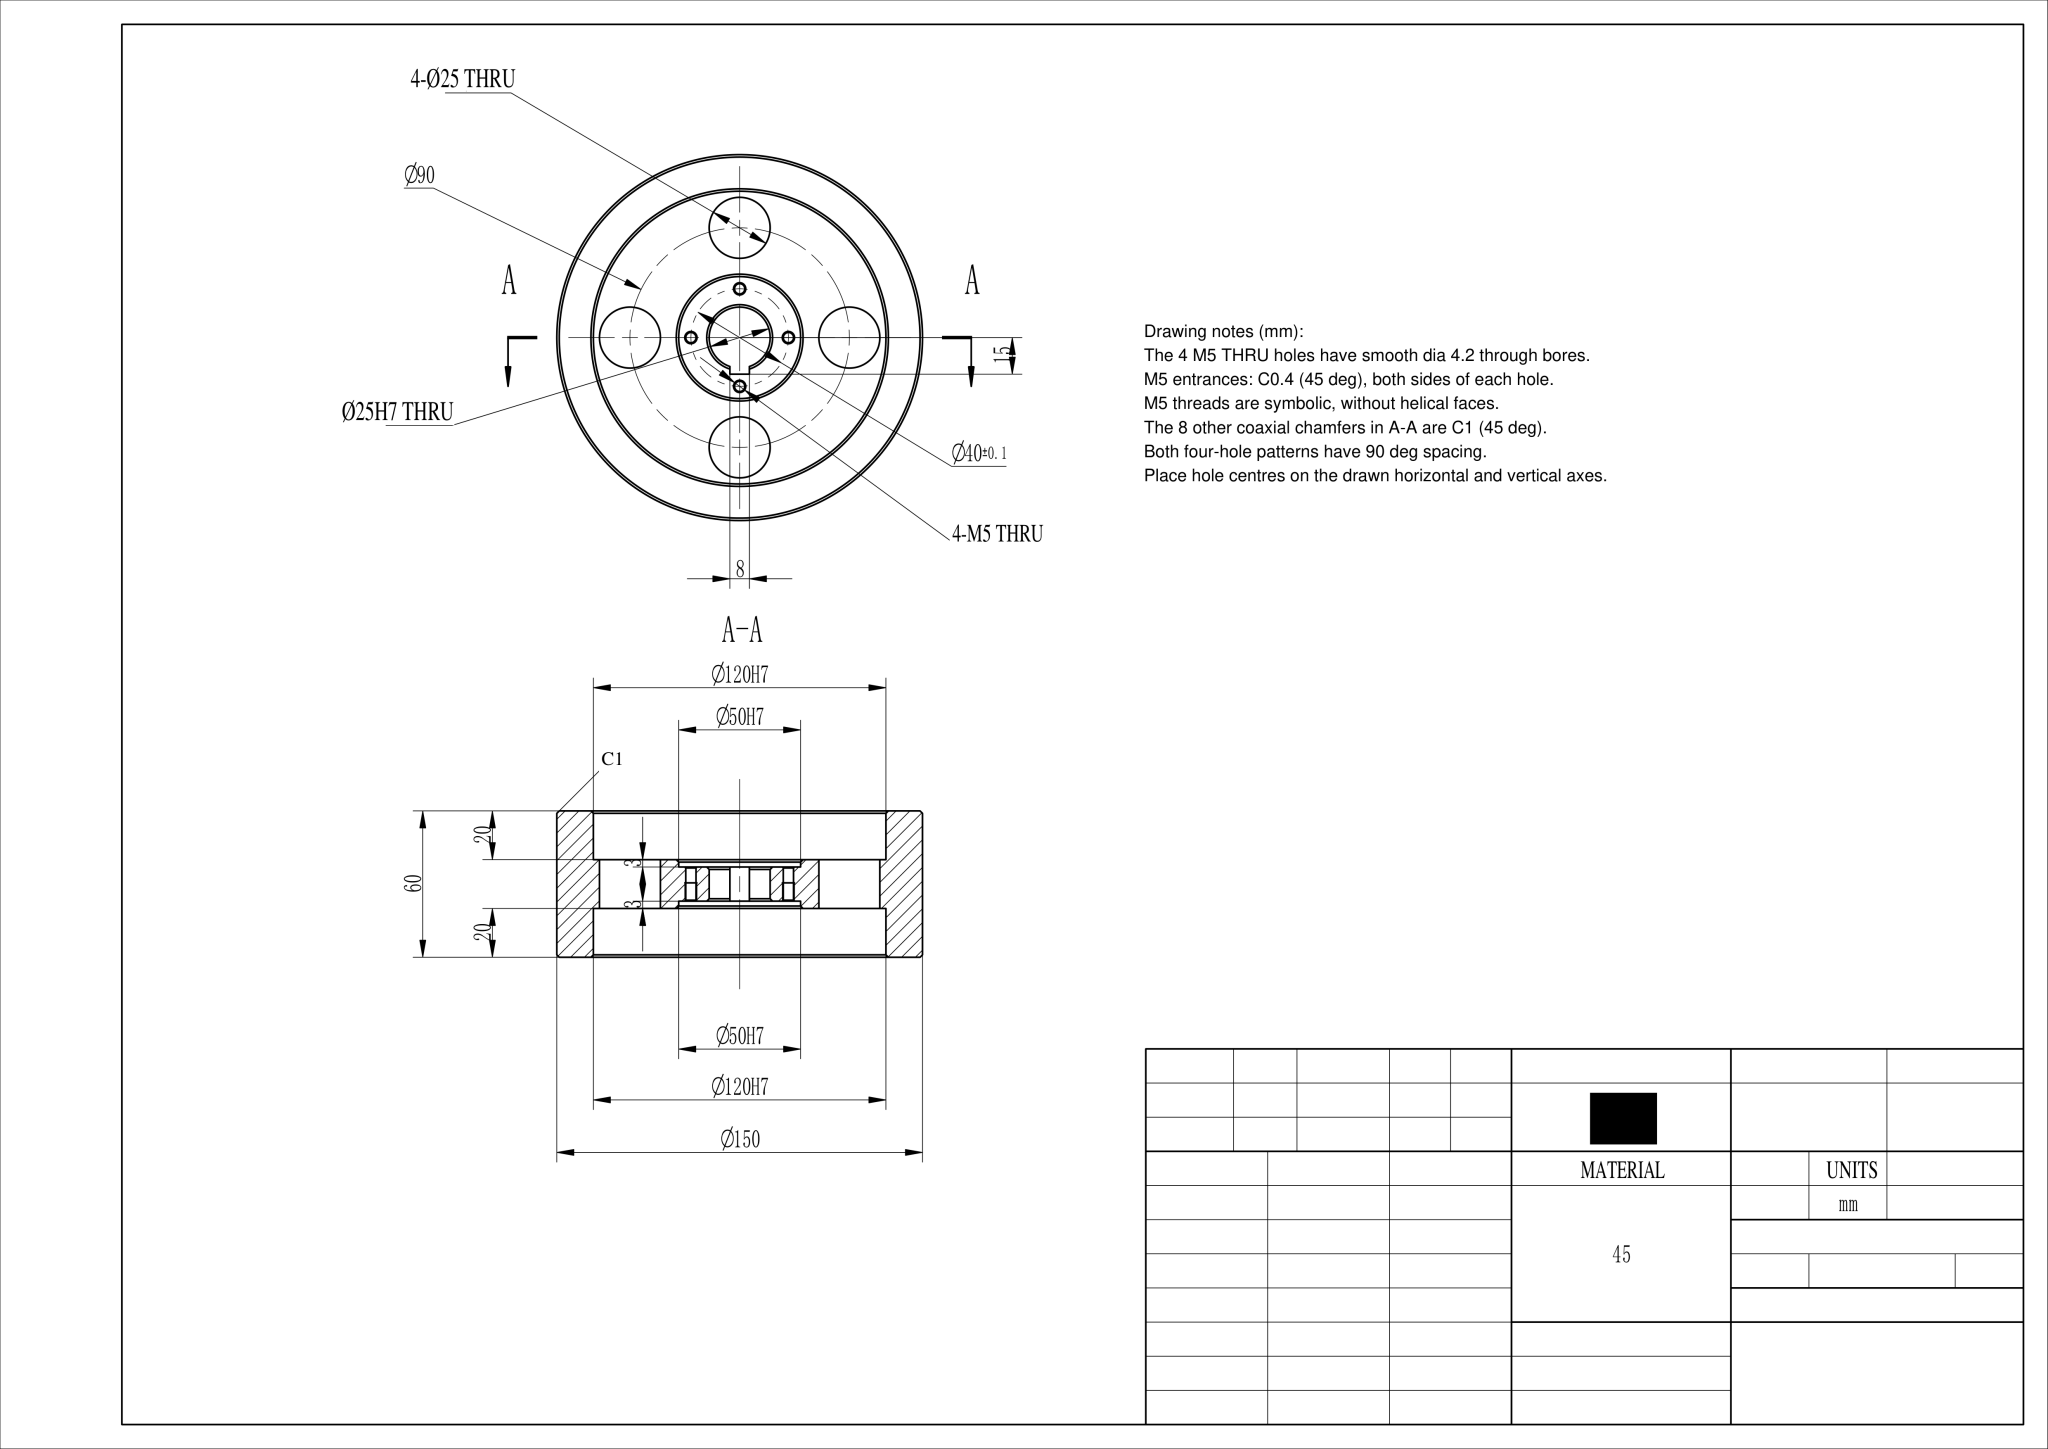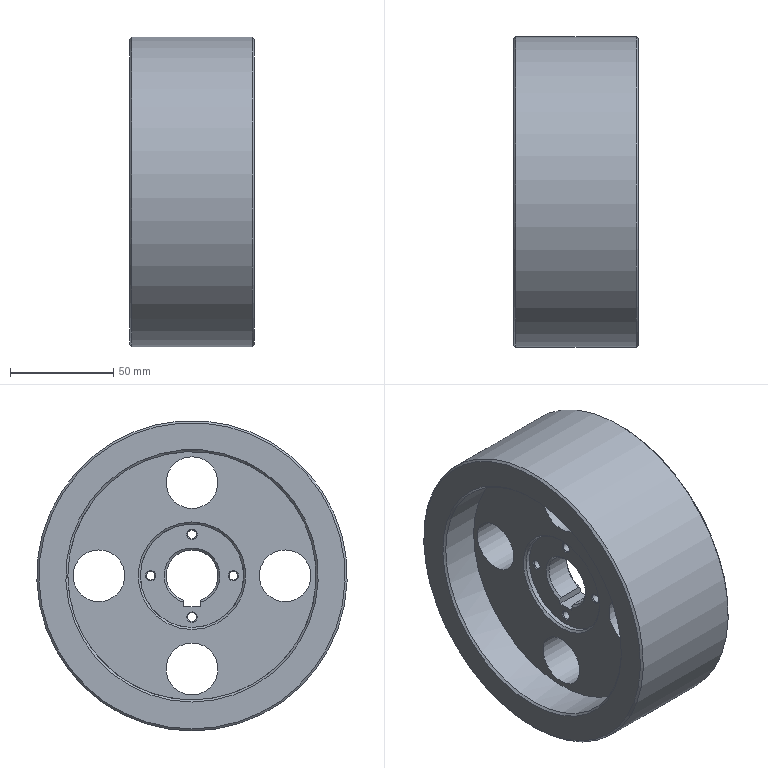Part | NX | mm | 1 solid | 39 faces | box 60 x 150 x 150 mm | volume 547806 mm3 | cone 16 | cylinder 14 | plane 9 | commonest cylinder face diameters 25 x5 4.2 x4 120 x2 50 x2 150 x1
STEP:
#1=CARTESIAN_POINT('',(0.,0.,0.));
#2=DIRECTION('',(0.,0.,1.));
#3=DIRECTION('',(1.,0.,0.));
#4=AXIS2_PLACEMENT_3D('',#1,#2,#3);
#5=(LENGTH_UNIT()NAMED_UNIT(*)SI_UNIT(.MILLI.,.METRE.));
#6=UNCERTAINTY_MEASURE_WITH_UNIT(LENGTH_MEASURE(0.0508),#5,'','');
#7=(NAMED_UNIT(*)PLANE_ANGLE_UNIT()SI_UNIT($,.RADIAN.));
#8=PLANE_ANGLE_MEASURE_WITH_UNIT(PLANE_ANGLE_MEASURE(0.01745),#7);
#9=DIMENSIONAL_EXPONENTS(0.,0.,0.,0.,0.,0.,0.);
#10=(CONVERSION_BASED_UNIT('',#8)NAMED_UNIT(#9)PLANE_ANGLE_UNIT());
#11=(NAMED_UNIT(*)SI_UNIT($,.STERADIAN.)SOLID_ANGLE_UNIT());
#12=(GEOMETRIC_REPRESENTATION_CONTEXT(3)GLOBAL_UNCERTAINTY_ASSIGNED_CONTEXT((#6))GLOBAL_UNIT_ASSIGNED_CONTEXT((#5,#10,#11))REPRESENTATION_CONTEXT('',''));
#13=SHAPE_REPRESENTATION('',(#4),#12);
#14=CARTESIAN_POINT('',(-29.,0.,-75.));
#15=VERTEX_POINT('',#14);
#16=CARTESIAN_POINT('',(-29.,0.,0.));
#17=DIRECTION('',(1.,0.,0.));
#18=DIRECTION('',(0.,0.,-1.));
#19=AXIS2_PLACEMENT_3D('',#16,#17,#18);
#20=CIRCLE('',#19,75.);
#21=EDGE_CURVE('',#15,#15,#20,.T.);
#22=ORIENTED_EDGE('',*,*,#21,.T.);
#23=EDGE_LOOP('',(#22));
#24=FACE_BOUND('',#23,.T.);
#25=CARTESIAN_POINT('',(29.,0.,-75.));
#26=VERTEX_POINT('',#25);
#27=CARTESIAN_POINT('',(29.,0.,0.));
#28=DIRECTION('',(-1.,0.,0.));
#29=DIRECTION('',(0.,0.,-1.));
#30=AXIS2_PLACEMENT_3D('',#27,#28,#29);
#31=CIRCLE('',#30,75.);
#32=EDGE_CURVE('',#26,#26,#31,.T.);
#33=ORIENTED_EDGE('',*,*,#32,.T.);
#34=EDGE_LOOP('',(#33));
#35=FACE_BOUND('',#34,.T.);
#36=CARTESIAN_POINT('',(30.,0.,0.));
#37=DIRECTION('',(-1.,0.,0.));
#38=DIRECTION('',(0.,0.,1.));
#39=AXIS2_PLACEMENT_3D('',#36,#37,#38);
#40=CYLINDRICAL_SURFACE('',#39,75.);
#41=ADVANCED_FACE('',(#24,#35),#40,.T.);
#42=CARTESIAN_POINT('',(30.,0.,-61.));
#43=VERTEX_POINT('',#42);
#44=CARTESIAN_POINT('',(30.,0.,0.));
#45=DIRECTION('',(-1.,0.,0.));
#46=DIRECTION('',(0.,0.,-1.));
#47=AXIS2_PLACEMENT_3D('',#44,#45,#46);
#48=CIRCLE('',#47,61.);
#49=EDGE_CURVE('',#43,#43,#48,.T.);
#50=ORIENTED_EDGE('',*,*,#49,.T.);
#51=EDGE_LOOP('',(#50));
#52=FACE_BOUND('',#51,.T.);
#53=CARTESIAN_POINT('',(30.,0.,-74.));
#54=VERTEX_POINT('',#53);
#55=CARTESIAN_POINT('',(30.,0.,0.));
#56=DIRECTION('',(1.,0.,0.));
#57=DIRECTION('',(0.,0.,-1.));
#58=AXIS2_PLACEMENT_3D('',#55,#56,#57);
#59=CIRCLE('',#58,74.);
#60=EDGE_CURVE('',#54,#54,#59,.T.);
#61=ORIENTED_EDGE('',*,*,#60,.T.);
#62=EDGE_LOOP('',(#61));
#63=FACE_BOUND('',#62,.T.);
#64=CARTESIAN_POINT('',(30.,0.,0.));
#65=DIRECTION('',(1.,0.,0.));
#66=DIRECTION('',(0.,0.,-1.));
#67=AXIS2_PLACEMENT_3D('',#64,#65,#66);
#68=PLANE('',#67);
#69=ADVANCED_FACE('',(#52,#63),#68,.T.);
#70=CARTESIAN_POINT('',(-30.,0.,-61.));
#71=VERTEX_POINT('',#70);
#72=CARTESIAN_POINT('',(-30.,0.,0.));
#73=DIRECTION('',(1.,0.,0.));
#74=DIRECTION('',(0.,0.,-1.));
#75=AXIS2_PLACEMENT_3D('',#72,#73,#74);
#76=CIRCLE('',#75,61.);
#77=EDGE_CURVE('',#71,#71,#76,.T.);
#78=ORIENTED_EDGE('',*,*,#77,.T.);
#79=EDGE_LOOP('',(#78));
#80=FACE_BOUND('',#79,.T.);
#81=CARTESIAN_POINT('',(-30.,0.,-74.));
#82=VERTEX_POINT('',#81);
#83=CARTESIAN_POINT('',(-30.,0.,0.));
#84=DIRECTION('',(-1.,0.,0.));
#85=DIRECTION('',(0.,0.,-1.));
#86=AXIS2_PLACEMENT_3D('',#83,#84,#85);
#87=CIRCLE('',#86,74.);
#88=EDGE_CURVE('',#82,#82,#87,.T.);
#89=ORIENTED_EDGE('',*,*,#88,.T.);
#90=EDGE_LOOP('',(#89));
#91=FACE_BOUND('',#90,.T.);
#92=CARTESIAN_POINT('',(-30.,0.,0.));
#93=DIRECTION('',(1.,0.,0.));
#94=DIRECTION('',(0.,0.,-1.));
#95=AXIS2_PLACEMENT_3D('',#92,#93,#94);
#96=PLANE('',#95);
#97=ADVANCED_FACE('',(#80,#91),#96,.F.);
#98=CARTESIAN_POINT('',(29.,0.,-60.));
#99=VERTEX_POINT('',#98);
#100=CARTESIAN_POINT('',(29.,0.,0.));
#101=DIRECTION('',(1.,0.,0.));
#102=DIRECTION('',(0.,0.,-1.));
#103=AXIS2_PLACEMENT_3D('',#100,#101,#102);
#104=CIRCLE('',#103,60.);
#105=EDGE_CURVE('',#99,#99,#104,.T.);
#106=ORIENTED_EDGE('',*,*,#105,.T.);
#107=EDGE_LOOP('',(#106));
#108=FACE_BOUND('',#107,.T.);
#109=CARTESIAN_POINT('',(10.,60.,-0.));
#110=VERTEX_POINT('',#109);
#111=CARTESIAN_POINT('',(10.,0.,0.));
#112=DIRECTION('',(-1.,0.,0.));
#113=DIRECTION('',(0.,1.,-0.));
#114=AXIS2_PLACEMENT_3D('',#111,#112,#113);
#115=CIRCLE('',#114,60.);
#116=EDGE_CURVE('',#110,#110,#115,.T.);
#117=ORIENTED_EDGE('',*,*,#116,.T.);
#118=EDGE_LOOP('',(#117));
#119=FACE_BOUND('',#118,.T.);
#120=CARTESIAN_POINT('',(10.,0.,0.));
#121=DIRECTION('',(1.,0.,0.));
#122=DIRECTION('',(0.,0.,-1.));
#123=AXIS2_PLACEMENT_3D('',#120,#121,#122);
#124=CYLINDRICAL_SURFACE('',#123,60.);
#125=ADVANCED_FACE('',(#108,#119),#124,.F.);
#126=CARTESIAN_POINT('',(10.,0.,-26.));
#127=VERTEX_POINT('',#126);
#128=CARTESIAN_POINT('',(10.,0.,0.));
#129=DIRECTION('',(-1.,0.,0.));
#130=DIRECTION('',(0.,0.,-1.));
#131=AXIS2_PLACEMENT_3D('',#128,#129,#130);
#132=CIRCLE('',#131,26.);
#133=EDGE_CURVE('',#127,#127,#132,.T.);
#134=ORIENTED_EDGE('',*,*,#133,.T.);
#135=EDGE_LOOP('',(#134));
#136=FACE_BOUND('',#135,.T.);
#137=CARTESIAN_POINT('',(10.,-45.,12.5));
#138=VERTEX_POINT('',#137);
#139=CARTESIAN_POINT('',(10.,-45.,-0.));
#140=DIRECTION('',(-1.,0.,0.));
#141=DIRECTION('',(0.,0.,1.));
#142=AXIS2_PLACEMENT_3D('',#139,#140,#141);
#143=CIRCLE('',#142,12.5);
#144=EDGE_CURVE('',#138,#138,#143,.T.);
#145=ORIENTED_EDGE('',*,*,#144,.T.);
#146=EDGE_LOOP('',(#145));
#147=FACE_BOUND('',#146,.T.);
#148=CARTESIAN_POINT('',(10.,0.,-32.5));
#149=VERTEX_POINT('',#148);
#150=CARTESIAN_POINT('',(10.,0.,-45.));
#151=DIRECTION('',(-1.,0.,0.));
#152=DIRECTION('',(0.,0.,1.));
#153=AXIS2_PLACEMENT_3D('',#150,#151,#152);
#154=CIRCLE('',#153,12.5);
#155=EDGE_CURVE('',#149,#149,#154,.T.);
#156=ORIENTED_EDGE('',*,*,#155,.T.);
#157=EDGE_LOOP('',(#156));
#158=FACE_BOUND('',#157,.T.);
#159=CARTESIAN_POINT('',(10.,45.,12.5));
#160=VERTEX_POINT('',#159);
#161=CARTESIAN_POINT('',(10.,45.,0.));
#162=DIRECTION('',(-1.,0.,0.));
#163=DIRECTION('',(0.,0.,1.));
#164=AXIS2_PLACEMENT_3D('',#161,#162,#163);
#165=CIRCLE('',#164,12.5);
#166=EDGE_CURVE('',#160,#160,#165,.T.);
#167=ORIENTED_EDGE('',*,*,#166,.T.);
#168=EDGE_LOOP('',(#167));
#169=FACE_BOUND('',#168,.T.);
#170=CARTESIAN_POINT('',(10.,0.,57.5));
#171=VERTEX_POINT('',#170);
#172=CARTESIAN_POINT('',(10.,0.,45.));
#173=DIRECTION('',(-1.,0.,0.));
#174=DIRECTION('',(0.,0.,1.));
#175=AXIS2_PLACEMENT_3D('',#172,#173,#174);
#176=CIRCLE('',#175,12.5);
#177=EDGE_CURVE('',#171,#171,#176,.T.);
#178=ORIENTED_EDGE('',*,*,#177,.T.);
#179=EDGE_LOOP('',(#178));
#180=FACE_BOUND('',#179,.T.);
#181=ORIENTED_EDGE('',*,*,#116,.F.);
#182=EDGE_LOOP('',(#181));
#183=FACE_BOUND('',#182,.T.);
#184=CARTESIAN_POINT('',(10.,0.,0.));
#185=DIRECTION('',(1.,0.,0.));
#186=DIRECTION('',(0.,0.,-1.));
#187=AXIS2_PLACEMENT_3D('',#184,#185,#186);
#188=PLANE('',#187);
#189=ADVANCED_FACE('',(#136,#147,#158,#169,#180,#183),#188,.T.);
#190=CARTESIAN_POINT('',(-29.,0.,-60.));
#191=VERTEX_POINT('',#190);
#192=CARTESIAN_POINT('',(-29.,0.,0.));
#193=DIRECTION('',(-1.,0.,0.));
#194=DIRECTION('',(0.,0.,-1.));
#195=AXIS2_PLACEMENT_3D('',#192,#193,#194);
#196=CIRCLE('',#195,60.);
#197=EDGE_CURVE('',#191,#191,#196,.T.);
#198=ORIENTED_EDGE('',*,*,#197,.T.);
#199=EDGE_LOOP('',(#198));
#200=FACE_BOUND('',#199,.T.);
#201=CARTESIAN_POINT('',(-10.,60.,-0.));
#202=VERTEX_POINT('',#201);
#203=CARTESIAN_POINT('',(-10.,0.,0.));
#204=DIRECTION('',(-1.,0.,0.));
#205=DIRECTION('',(0.,1.,-0.));
#206=AXIS2_PLACEMENT_3D('',#203,#204,#205);
#207=CIRCLE('',#206,60.);
#208=EDGE_CURVE('',#202,#202,#207,.T.);
#209=ORIENTED_EDGE('',*,*,#208,.F.);
#210=EDGE_LOOP('',(#209));
#211=FACE_BOUND('',#210,.T.);
#212=CARTESIAN_POINT('',(-10.,0.,0.));
#213=DIRECTION('',(-1.,0.,0.));
#214=DIRECTION('',(0.,0.,1.));
#215=AXIS2_PLACEMENT_3D('',#212,#213,#214);
#216=CYLINDRICAL_SURFACE('',#215,60.);
#217=ADVANCED_FACE('',(#200,#211),#216,.F.);
#218=CARTESIAN_POINT('',(-10.,0.,-26.));
#219=VERTEX_POINT('',#218);
#220=CARTESIAN_POINT('',(-10.,0.,0.));
#221=DIRECTION('',(1.,0.,0.));
#222=DIRECTION('',(0.,0.,-1.));
#223=AXIS2_PLACEMENT_3D('',#220,#221,#222);
#224=CIRCLE('',#223,26.);
#225=EDGE_CURVE('',#219,#219,#224,.T.);
#226=ORIENTED_EDGE('',*,*,#225,.T.);
#227=EDGE_LOOP('',(#226));
#228=FACE_BOUND('',#227,.T.);
#229=CARTESIAN_POINT('',(-10.,-45.,-12.5));
#230=VERTEX_POINT('',#229);
#231=CARTESIAN_POINT('',(-10.,-45.,-0.));
#232=DIRECTION('',(1.,0.,0.));
#233=DIRECTION('',(0.,0.,-1.));
#234=AXIS2_PLACEMENT_3D('',#231,#232,#233);
#235=CIRCLE('',#234,12.5);
#236=EDGE_CURVE('',#230,#230,#235,.T.);
#237=ORIENTED_EDGE('',*,*,#236,.T.);
#238=EDGE_LOOP('',(#237));
#239=FACE_BOUND('',#238,.T.);
#240=CARTESIAN_POINT('',(-10.,0.,-57.5));
#241=VERTEX_POINT('',#240);
#242=CARTESIAN_POINT('',(-10.,0.,-45.));
#243=DIRECTION('',(1.,0.,0.));
#244=DIRECTION('',(0.,0.,-1.));
#245=AXIS2_PLACEMENT_3D('',#242,#243,#244);
#246=CIRCLE('',#245,12.5);
#247=EDGE_CURVE('',#241,#241,#246,.T.);
#248=ORIENTED_EDGE('',*,*,#247,.T.);
#249=EDGE_LOOP('',(#248));
#250=FACE_BOUND('',#249,.T.);
#251=CARTESIAN_POINT('',(-10.,45.,-12.5));
#252=VERTEX_POINT('',#251);
#253=CARTESIAN_POINT('',(-10.,45.,0.));
#254=DIRECTION('',(1.,0.,0.));
#255=DIRECTION('',(0.,0.,-1.));
#256=AXIS2_PLACEMENT_3D('',#253,#254,#255);
#257=CIRCLE('',#256,12.5);
#258=EDGE_CURVE('',#252,#252,#257,.T.);
#259=ORIENTED_EDGE('',*,*,#258,.T.);
#260=EDGE_LOOP('',(#259));
#261=FACE_BOUND('',#260,.T.);
#262=CARTESIAN_POINT('',(-10.,0.,32.5));
#263=VERTEX_POINT('',#262);
#264=CARTESIAN_POINT('',(-10.,0.,45.));
#265=DIRECTION('',(1.,0.,0.));
#266=DIRECTION('',(0.,0.,-1.));
#267=AXIS2_PLACEMENT_3D('',#264,#265,#266);
#268=CIRCLE('',#267,12.5);
#269=EDGE_CURVE('',#263,#263,#268,.T.);
#270=ORIENTED_EDGE('',*,*,#269,.T.);
#271=EDGE_LOOP('',(#270));
#272=FACE_BOUND('',#271,.T.);
#273=ORIENTED_EDGE('',*,*,#208,.T.);
#274=EDGE_LOOP('',(#273));
#275=FACE_BOUND('',#274,.T.);
#276=CARTESIAN_POINT('',(-10.,0.,0.));
#277=DIRECTION('',(1.,0.,0.));
#278=DIRECTION('',(0.,0.,-1.));
#279=AXIS2_PLACEMENT_3D('',#276,#277,#278);
#280=PLANE('',#279);
#281=ADVANCED_FACE('',(#228,#239,#250,#261,#272,#275),#280,.F.);
#282=ORIENTED_EDGE('',*,*,#177,.F.);
#283=EDGE_LOOP('',(#282));
#284=FACE_BOUND('',#283,.T.);
#285=ORIENTED_EDGE('',*,*,#269,.F.);
#286=EDGE_LOOP('',(#285));
#287=FACE_BOUND('',#286,.T.);
#288=CARTESIAN_POINT('',(10.,0.,45.));
#289=DIRECTION('',(-1.,0.,0.));
#290=DIRECTION('',(0.,0.,1.));
#291=AXIS2_PLACEMENT_3D('',#288,#289,#290);
#292=CYLINDRICAL_SURFACE('',#291,12.5);
#293=ADVANCED_FACE('',(#284,#287),#292,.F.);
#294=ORIENTED_EDGE('',*,*,#166,.F.);
#295=EDGE_LOOP('',(#294));
#296=FACE_BOUND('',#295,.T.);
#297=ORIENTED_EDGE('',*,*,#258,.F.);
#298=EDGE_LOOP('',(#297));
#299=FACE_BOUND('',#298,.T.);
#300=CARTESIAN_POINT('',(10.,45.,0.));
#301=DIRECTION('',(-1.,0.,0.));
#302=DIRECTION('',(0.,0.,1.));
#303=AXIS2_PLACEMENT_3D('',#300,#301,#302);
#304=CYLINDRICAL_SURFACE('',#303,12.5);
#305=ADVANCED_FACE('',(#296,#299),#304,.F.);
#306=ORIENTED_EDGE('',*,*,#155,.F.);
#307=EDGE_LOOP('',(#306));
#308=FACE_BOUND('',#307,.T.);
#309=ORIENTED_EDGE('',*,*,#247,.F.);
#310=EDGE_LOOP('',(#309));
#311=FACE_BOUND('',#310,.T.);
#312=CARTESIAN_POINT('',(10.,0.,-45.));
#313=DIRECTION('',(-1.,0.,0.));
#314=DIRECTION('',(0.,0.,1.));
#315=AXIS2_PLACEMENT_3D('',#312,#313,#314);
#316=CYLINDRICAL_SURFACE('',#315,12.5);
#317=ADVANCED_FACE('',(#308,#311),#316,.F.);
#318=ORIENTED_EDGE('',*,*,#144,.F.);
#319=EDGE_LOOP('',(#318));
#320=FACE_BOUND('',#319,.T.);
#321=ORIENTED_EDGE('',*,*,#236,.F.);
#322=EDGE_LOOP('',(#321));
#323=FACE_BOUND('',#322,.T.);
#324=CARTESIAN_POINT('',(10.,-45.,-0.));
#325=DIRECTION('',(-1.,0.,0.));
#326=DIRECTION('',(0.,0.,1.));
#327=AXIS2_PLACEMENT_3D('',#324,#325,#326);
#328=CYLINDRICAL_SURFACE('',#327,12.5);
#329=ADVANCED_FACE('',(#320,#323),#328,.F.);
#330=CARTESIAN_POINT('',(9.,0.,-25.));
#331=VERTEX_POINT('',#330);
#332=CARTESIAN_POINT('',(9.,0.,0.));
#333=DIRECTION('',(1.,0.,0.));
#334=DIRECTION('',(0.,0.,-1.));
#335=AXIS2_PLACEMENT_3D('',#332,#333,#334);
#336=CIRCLE('',#335,25.);
#337=EDGE_CURVE('',#331,#331,#336,.T.);
#338=ORIENTED_EDGE('',*,*,#337,.T.);
#339=EDGE_LOOP('',(#338));
#340=FACE_BOUND('',#339,.T.);
#341=CARTESIAN_POINT('',(7.,25.,-0.));
#342=VERTEX_POINT('',#341);
#343=CARTESIAN_POINT('',(7.,0.,0.));
#344=DIRECTION('',(-1.,0.,0.));
#345=DIRECTION('',(0.,1.,-0.));
#346=AXIS2_PLACEMENT_3D('',#343,#344,#345);
#347=CIRCLE('',#346,25.);
#348=EDGE_CURVE('',#342,#342,#347,.T.);
#349=ORIENTED_EDGE('',*,*,#348,.T.);
#350=EDGE_LOOP('',(#349));
#351=FACE_BOUND('',#350,.T.);
#352=CARTESIAN_POINT('',(7.,0.,0.));
#353=DIRECTION('',(1.,0.,0.));
#354=DIRECTION('',(0.,0.,-1.));
#355=AXIS2_PLACEMENT_3D('',#352,#353,#354);
#356=CYLINDRICAL_SURFACE('',#355,25.);
#357=ADVANCED_FACE('',(#340,#351),#356,.F.);
#358=CARTESIAN_POINT('',(7.,4.,-15.));
#359=VERTEX_POINT('',#358);
#360=CARTESIAN_POINT('',(7.,4.,-12.894));
#361=VERTEX_POINT('',#360);
#362=CARTESIAN_POINT('',(7.,4.,0.));
#363=DIRECTION('',(0.,-0.,1.));
#364=VECTOR('',#363,1.);
#365=LINE('',#362,#364);
#366=EDGE_CURVE('',#359,#361,#365,.T.);
#367=ORIENTED_EDGE('',*,*,#366,.F.);
#368=CARTESIAN_POINT('',(7.,-4.,-15.));
#369=VERTEX_POINT('',#368);
#370=CARTESIAN_POINT('',(7.,0.,-15.));
#371=DIRECTION('',(0.,1.,0.));
#372=VECTOR('',#371,1.);
#373=LINE('',#370,#372);
#374=EDGE_CURVE('',#369,#359,#373,.T.);
#375=ORIENTED_EDGE('',*,*,#374,.F.);
#376=CARTESIAN_POINT('',(7.,-4.,-12.894));
#377=VERTEX_POINT('',#376);
#378=CARTESIAN_POINT('',(7.,-4.,0.));
#379=DIRECTION('',(0.,-0.,-1.));
#380=VECTOR('',#379,1.);
#381=LINE('',#378,#380);
#382=EDGE_CURVE('',#377,#369,#381,.T.);
#383=ORIENTED_EDGE('',*,*,#382,.F.);
#384=CARTESIAN_POINT('',(7.,0.,0.));
#385=DIRECTION('',(-1.,0.,0.));
#386=DIRECTION('',(0.,0.,-1.));
#387=AXIS2_PLACEMENT_3D('',#384,#385,#386);
#388=CIRCLE('',#387,13.5);
#389=EDGE_CURVE('',#377,#361,#388,.T.);
#390=ORIENTED_EDGE('',*,*,#389,.T.);
#391=EDGE_LOOP('',(#367,#375,#383,#390));
#392=FACE_BOUND('',#391,.T.);
#393=CARTESIAN_POINT('',(7.,-20.,-2.5));
#394=VERTEX_POINT('',#393);
#395=CARTESIAN_POINT('',(7.,-20.,0.));
#396=DIRECTION('',(-1.,0.,0.));
#397=DIRECTION('',(0.,0.,-1.));
#398=AXIS2_PLACEMENT_3D('',#395,#396,#397);
#399=CIRCLE('',#398,2.5);
#400=EDGE_CURVE('',#394,#394,#399,.T.);
#401=ORIENTED_EDGE('',*,*,#400,.T.);
#402=EDGE_LOOP('',(#401));
#403=FACE_BOUND('',#402,.T.);
#404=CARTESIAN_POINT('',(7.,0.,17.5));
#405=VERTEX_POINT('',#404);
#406=CARTESIAN_POINT('',(7.,0.,20.));
#407=DIRECTION('',(-1.,0.,0.));
#408=DIRECTION('',(0.,0.,-1.));
#409=AXIS2_PLACEMENT_3D('',#406,#407,#408);
#410=CIRCLE('',#409,2.5);
#411=EDGE_CURVE('',#405,#405,#410,.T.);
#412=ORIENTED_EDGE('',*,*,#411,.T.);
#413=EDGE_LOOP('',(#412));
#414=FACE_BOUND('',#413,.T.);
#415=CARTESIAN_POINT('',(7.,20.,-2.5));
#416=VERTEX_POINT('',#415);
#417=CARTESIAN_POINT('',(7.,20.,-0.));
#418=DIRECTION('',(-1.,0.,0.));
#419=DIRECTION('',(0.,0.,-1.));
#420=AXIS2_PLACEMENT_3D('',#417,#418,#419);
#421=CIRCLE('',#420,2.5);
#422=EDGE_CURVE('',#416,#416,#421,.T.);
#423=ORIENTED_EDGE('',*,*,#422,.T.);
#424=EDGE_LOOP('',(#423));
#425=FACE_BOUND('',#424,.T.);
#426=CARTESIAN_POINT('',(7.,0.,-22.5));
#427=VERTEX_POINT('',#426);
#428=CARTESIAN_POINT('',(7.,0.,-20.));
#429=DIRECTION('',(-1.,0.,0.));
#430=DIRECTION('',(0.,0.,-1.));
#431=AXIS2_PLACEMENT_3D('',#428,#429,#430);
#432=CIRCLE('',#431,2.5);
#433=EDGE_CURVE('',#427,#427,#432,.T.);
#434=ORIENTED_EDGE('',*,*,#433,.T.);
#435=EDGE_LOOP('',(#434));
#436=FACE_BOUND('',#435,.T.);
#437=ORIENTED_EDGE('',*,*,#348,.F.);
#438=EDGE_LOOP('',(#437));
#439=FACE_BOUND('',#438,.T.);
#440=CARTESIAN_POINT('',(7.,0.,0.));
#441=DIRECTION('',(1.,0.,0.));
#442=DIRECTION('',(0.,0.,-1.));
#443=AXIS2_PLACEMENT_3D('',#440,#441,#442);
#444=PLANE('',#443);
#445=ADVANCED_FACE('',(#392,#403,#414,#425,#436,#439),#444,.T.);
#446=CARTESIAN_POINT('',(-9.,0.,-25.));
#447=VERTEX_POINT('',#446);
#448=CARTESIAN_POINT('',(-9.,0.,0.));
#449=DIRECTION('',(-1.,0.,0.));
#450=DIRECTION('',(0.,0.,-1.));
#451=AXIS2_PLACEMENT_3D('',#448,#449,#450);
#452=CIRCLE('',#451,25.);
#453=EDGE_CURVE('',#447,#447,#452,.T.);
#454=ORIENTED_EDGE('',*,*,#453,.T.);
#455=EDGE_LOOP('',(#454));
#456=FACE_BOUND('',#455,.T.);
#457=CARTESIAN_POINT('',(-7.,25.,-0.));
#458=VERTEX_POINT('',#457);
#459=CARTESIAN_POINT('',(-7.,0.,0.));
#460=DIRECTION('',(-1.,0.,0.));
#461=DIRECTION('',(0.,1.,-0.));
#462=AXIS2_PLACEMENT_3D('',#459,#460,#461);
#463=CIRCLE('',#462,25.);
#464=EDGE_CURVE('',#458,#458,#463,.T.);
#465=ORIENTED_EDGE('',*,*,#464,.F.);
#466=EDGE_LOOP('',(#465));
#467=FACE_BOUND('',#466,.T.);
#468=CARTESIAN_POINT('',(-7.,0.,0.));
#469=DIRECTION('',(-1.,0.,0.));
#470=DIRECTION('',(0.,0.,1.));
#471=AXIS2_PLACEMENT_3D('',#468,#469,#470);
#472=CYLINDRICAL_SURFACE('',#471,25.);
#473=ADVANCED_FACE('',(#456,#467),#472,.F.);
#474=CARTESIAN_POINT('',(-7.,-20.,-2.5));
#475=VERTEX_POINT('',#474);
#476=CARTESIAN_POINT('',(-7.,-20.,0.));
#477=DIRECTION('',(1.,0.,0.));
#478=DIRECTION('',(0.,0.,-1.));
#479=AXIS2_PLACEMENT_3D('',#476,#477,#478);
#480=CIRCLE('',#479,2.5);
#481=EDGE_CURVE('',#475,#475,#480,.T.);
#482=ORIENTED_EDGE('',*,*,#481,.T.);
#483=EDGE_LOOP('',(#482));
#484=FACE_BOUND('',#483,.T.);
#485=CARTESIAN_POINT('',(-7.,0.,17.5));
#486=VERTEX_POINT('',#485);
#487=CARTESIAN_POINT('',(-7.,0.,20.));
#488=DIRECTION('',(1.,0.,0.));
#489=DIRECTION('',(0.,0.,-1.));
#490=AXIS2_PLACEMENT_3D('',#487,#488,#489);
#491=CIRCLE('',#490,2.5);
#492=EDGE_CURVE('',#486,#486,#491,.T.);
#493=ORIENTED_EDGE('',*,*,#492,.T.);
#494=EDGE_LOOP('',(#493));
#495=FACE_BOUND('',#494,.T.);
#496=CARTESIAN_POINT('',(-7.,20.,-2.5));
#497=VERTEX_POINT('',#496);
#498=CARTESIAN_POINT('',(-7.,20.,-0.));
#499=DIRECTION('',(1.,0.,0.));
#500=DIRECTION('',(0.,0.,-1.));
#501=AXIS2_PLACEMENT_3D('',#498,#499,#500);
#502=CIRCLE('',#501,2.5);
#503=EDGE_CURVE('',#497,#497,#502,.T.);
#504=ORIENTED_EDGE('',*,*,#503,.T.);
#505=EDGE_LOOP('',(#504));
#506=FACE_BOUND('',#505,.T.);
#507=CARTESIAN_POINT('',(-7.,0.,-22.5));
#508=VERTEX_POINT('',#507);
#509=CARTESIAN_POINT('',(-7.,0.,-20.));
#510=DIRECTION('',(1.,0.,0.));
#511=DIRECTION('',(0.,0.,-1.));
#512=AXIS2_PLACEMENT_3D('',#509,#510,#511);
#513=CIRCLE('',#512,2.5);
#514=EDGE_CURVE('',#508,#508,#513,.T.);
#515=ORIENTED_EDGE('',*,*,#514,.T.);
#516=EDGE_LOOP('',(#515));
#517=FACE_BOUND('',#516,.T.);
#518=CARTESIAN_POINT('',(-7.,-4.,-15.));
#519=VERTEX_POINT('',#518);
#520=CARTESIAN_POINT('',(-7.,4.,-15.));
#521=VERTEX_POINT('',#520);
#522=CARTESIAN_POINT('',(-7.,0.,-15.));
#523=DIRECTION('',(0.,1.,0.));
#524=VECTOR('',#523,1.);
#525=LINE('',#522,#524);
#526=EDGE_CURVE('',#519,#521,#525,.T.);
#527=ORIENTED_EDGE('',*,*,#526,.T.);
#528=CARTESIAN_POINT('',(-7.,4.,-12.894));
#529=VERTEX_POINT('',#528);
#530=CARTESIAN_POINT('',(-7.,4.,0.));
#531=DIRECTION('',(0.,-0.,1.));
#532=VECTOR('',#531,1.);
#533=LINE('',#530,#532);
#534=EDGE_CURVE('',#521,#529,#533,.T.);
#535=ORIENTED_EDGE('',*,*,#534,.T.);
#536=CARTESIAN_POINT('',(-7.,-4.,-12.894));
#537=VERTEX_POINT('',#536);
#538=CARTESIAN_POINT('',(-7.,0.,0.));
#539=DIRECTION('',(1.,0.,0.));
#540=DIRECTION('',(0.,0.,-1.));
#541=AXIS2_PLACEMENT_3D('',#538,#539,#540);
#542=CIRCLE('',#541,13.5);
#543=EDGE_CURVE('',#529,#537,#542,.T.);
#544=ORIENTED_EDGE('',*,*,#543,.T.);
#545=CARTESIAN_POINT('',(-7.,-4.,0.));
#546=DIRECTION('',(0.,-0.,-1.));
#547=VECTOR('',#546,1.);
#548=LINE('',#545,#547);
#549=EDGE_CURVE('',#537,#519,#548,.T.);
#550=ORIENTED_EDGE('',*,*,#549,.T.);
#551=EDGE_LOOP('',(#527,#535,#544,#550));
#552=FACE_BOUND('',#551,.T.);
#553=ORIENTED_EDGE('',*,*,#464,.T.);
#554=EDGE_LOOP('',(#553));
#555=FACE_BOUND('',#554,.T.);
#556=CARTESIAN_POINT('',(-7.,0.,0.));
#557=DIRECTION('',(1.,0.,0.));
#558=DIRECTION('',(0.,0.,-1.));
#559=AXIS2_PLACEMENT_3D('',#556,#557,#558);
#560=PLANE('',#559);
#561=ADVANCED_FACE('',(#484,#495,#506,#517,#552,#555),#560,.F.);
#562=CARTESIAN_POINT('',(-6.,-4.,-11.843));
#563=VERTEX_POINT('',#562);
#564=CARTESIAN_POINT('',(-6.,4.,-11.843));
#565=VERTEX_POINT('',#564);
#566=CARTESIAN_POINT('',(-6.,0.,0.));
#567=DIRECTION('',(-1.,0.,0.));
#568=DIRECTION('',(0.,0.,-1.));
#569=AXIS2_PLACEMENT_3D('',#566,#567,#568);
#570=CIRCLE('',#569,12.5);
#571=EDGE_CURVE('',#563,#565,#570,.T.);
#572=ORIENTED_EDGE('',*,*,#571,.T.);
#573=CARTESIAN_POINT('',(6.,4.,-11.843));
#574=VERTEX_POINT('',#573);
#575=CARTESIAN_POINT('',(-39.,4.,-11.843));
#576=DIRECTION('',(1.,0.,0.));
#577=VECTOR('',#576,1.);
#578=LINE('',#575,#577);
#579=EDGE_CURVE('',#565,#574,#578,.T.);
#580=ORIENTED_EDGE('',*,*,#579,.T.);
#581=CARTESIAN_POINT('',(6.,-4.,-11.843));
#582=VERTEX_POINT('',#581);
#583=CARTESIAN_POINT('',(6.,0.,0.));
#584=DIRECTION('',(1.,0.,0.));
#585=DIRECTION('',(0.,0.,-1.));
#586=AXIS2_PLACEMENT_3D('',#583,#584,#585);
#587=CIRCLE('',#586,12.5);
#588=EDGE_CURVE('',#574,#582,#587,.T.);
#589=ORIENTED_EDGE('',*,*,#588,.T.);
#590=CARTESIAN_POINT('',(-39.,-4.,-11.843));
#591=DIRECTION('',(-1.,0.,0.));
#592=VECTOR('',#591,1.);
#593=LINE('',#590,#592);
#594=EDGE_CURVE('',#582,#563,#593,.T.);
#595=ORIENTED_EDGE('',*,*,#594,.T.);
#596=EDGE_LOOP('',(#572,#580,#589,#595));
#597=FACE_OUTER_BOUND('',#596,.T.);
#598=CARTESIAN_POINT('',(-39.,0.,0.));
#599=DIRECTION('',(1.,0.,0.));
#600=DIRECTION('',(0.,0.,-1.));
#601=AXIS2_PLACEMENT_3D('',#598,#599,#600);
#602=CYLINDRICAL_SURFACE('',#601,12.5);
#603=ADVANCED_FACE('',(#597),#602,.F.);
#604=CARTESIAN_POINT('',(7.,4.,-12.894));
#605=CARTESIAN_POINT('',(6.751,4.,-12.633));
#606=CARTESIAN_POINT('',(6.501,4.,-12.371));
#607=CARTESIAN_POINT('',(6.253,4.,-12.109));
#608=CARTESIAN_POINT('',(6.168,4.,-12.02));
#609=CARTESIAN_POINT('',(6.084,4.,-11.932));
#610=CARTESIAN_POINT('',(6.,4.,-11.843));
#611=B_SPLINE_CURVE_WITH_KNOTS('',3,(#604,#605,#606,#607,#608,#609,#610),.UNSPECIFIED.,.F.,.F.,(4,3,4),(0.,0.7468,1.),.UNSPECIFIED.);
#612=EDGE_CURVE('',#361,#574,#611,.T.);
#613=ORIENTED_EDGE('',*,*,#612,.F.);
#614=ORIENTED_EDGE('',*,*,#389,.F.);
#615=CARTESIAN_POINT('',(6.,-4.,-11.843));
#616=CARTESIAN_POINT('',(6.084,-4.,-11.932));
#617=CARTESIAN_POINT('',(6.168,-4.,-12.02));
#618=CARTESIAN_POINT('',(6.253,-4.,-12.109));
#619=CARTESIAN_POINT('',(6.501,-4.,-12.371));
#620=CARTESIAN_POINT('',(6.751,-4.,-12.633));
#621=CARTESIAN_POINT('',(7.,-4.,-12.894));
#622=B_SPLINE_CURVE_WITH_KNOTS('',3,(#615,#616,#617,#618,#619,#620,#621),.UNSPECIFIED.,.F.,.F.,(4,3,4),(0.,0.2532,1.),.UNSPECIFIED.);
#623=EDGE_CURVE('',#582,#377,#622,.T.);
#624=ORIENTED_EDGE('',*,*,#623,.F.);
#625=ORIENTED_EDGE('',*,*,#588,.F.);
#626=EDGE_LOOP('',(#613,#614,#624,#625));
#627=FACE_OUTER_BOUND('',#626,.T.);
#628=CARTESIAN_POINT('',(6.,0.,0.));
#629=DIRECTION('',(1.,0.,0.));
#630=DIRECTION('',(0.,0.,-1.));
#631=AXIS2_PLACEMENT_3D('',#628,#629,#630);
#632=CONICAL_SURFACE('',#631,12.5,45.);
#633=ADVANCED_FACE('',(#627),#632,.F.);
#634=CARTESIAN_POINT('',(-6.,4.,-11.843));
#635=CARTESIAN_POINT('',(-6.084,4.,-11.932));
#636=CARTESIAN_POINT('',(-6.168,4.,-12.02));
#637=CARTESIAN_POINT('',(-6.253,4.,-12.109));
#638=CARTESIAN_POINT('',(-6.501,4.,-12.371));
#639=CARTESIAN_POINT('',(-6.751,4.,-12.633));
#640=CARTESIAN_POINT('',(-7.,4.,-12.894));
#641=B_SPLINE_CURVE_WITH_KNOTS('',3,(#634,#635,#636,#637,#638,#639,#640),.UNSPECIFIED.,.F.,.F.,(4,3,4),(0.,0.2532,1.),.UNSPECIFIED.);
#642=EDGE_CURVE('',#565,#529,#641,.T.);
#643=ORIENTED_EDGE('',*,*,#642,.F.);
#644=ORIENTED_EDGE('',*,*,#571,.F.);
#645=CARTESIAN_POINT('',(-7.,-4.,-12.894));
#646=CARTESIAN_POINT('',(-6.751,-4.,-12.633));
#647=CARTESIAN_POINT('',(-6.501,-4.,-12.371));
#648=CARTESIAN_POINT('',(-6.253,-4.,-12.109));
#649=CARTESIAN_POINT('',(-6.168,-4.,-12.02));
#650=CARTESIAN_POINT('',(-6.084,-4.,-11.932));
#651=CARTESIAN_POINT('',(-6.,-4.,-11.843));
#652=B_SPLINE_CURVE_WITH_KNOTS('',3,(#645,#646,#647,#648,#649,#650,#651),.UNSPECIFIED.,.F.,.F.,(4,3,4),(0.,0.7468,1.),.UNSPECIFIED.);
#653=EDGE_CURVE('',#537,#563,#652,.T.);
#654=ORIENTED_EDGE('',*,*,#653,.F.);
#655=ORIENTED_EDGE('',*,*,#543,.F.);
#656=EDGE_LOOP('',(#643,#644,#654,#655));
#657=FACE_OUTER_BOUND('',#656,.T.);
#658=CARTESIAN_POINT('',(-7.,0.,0.));
#659=DIRECTION('',(-1.,0.,0.));
#660=DIRECTION('',(0.,0.,1.));
#661=AXIS2_PLACEMENT_3D('',#658,#659,#660);
#662=CONICAL_SURFACE('',#661,13.5,45.);
#663=ADVANCED_FACE('',(#657),#662,.F.);
#664=ORIENTED_EDGE('',*,*,#32,.F.);
#665=EDGE_LOOP('',(#664));
#666=FACE_BOUND('',#665,.T.);
#667=ORIENTED_EDGE('',*,*,#60,.F.);
#668=EDGE_LOOP('',(#667));
#669=FACE_BOUND('',#668,.T.);
#670=CARTESIAN_POINT('',(30.,0.,0.));
#671=DIRECTION('',(-1.,0.,0.));
#672=DIRECTION('',(0.,0.,1.));
#673=AXIS2_PLACEMENT_3D('',#670,#671,#672);
#674=CONICAL_SURFACE('',#673,74.,45.);
#675=ADVANCED_FACE('',(#666,#669),#674,.T.);
#676=ORIENTED_EDGE('',*,*,#88,.F.);
#677=EDGE_LOOP('',(#676));
#678=FACE_BOUND('',#677,.T.);
#679=ORIENTED_EDGE('',*,*,#21,.F.);
#680=EDGE_LOOP('',(#679));
#681=FACE_BOUND('',#680,.T.);
#682=CARTESIAN_POINT('',(-29.,0.,0.));
#683=DIRECTION('',(1.,0.,0.));
#684=DIRECTION('',(-0.,0.,-1.));
#685=AXIS2_PLACEMENT_3D('',#682,#683,#684);
#686=CONICAL_SURFACE('',#685,75.,45.);
#687=ADVANCED_FACE('',(#678,#681),#686,.T.);
#688=ORIENTED_EDGE('',*,*,#197,.F.);
#689=EDGE_LOOP('',(#688));
#690=FACE_BOUND('',#689,.T.);
#691=ORIENTED_EDGE('',*,*,#77,.F.);
#692=EDGE_LOOP('',(#691));
#693=FACE_BOUND('',#692,.T.);
#694=CARTESIAN_POINT('',(-30.,0.,0.));
#695=DIRECTION('',(-1.,0.,0.));
#696=DIRECTION('',(-0.,0.,1.));
#697=AXIS2_PLACEMENT_3D('',#694,#695,#696);
#698=CONICAL_SURFACE('',#697,61.,45.);
#699=ADVANCED_FACE('',(#690,#693),#698,.F.);
#700=ORIENTED_EDGE('',*,*,#49,.F.);
#701=EDGE_LOOP('',(#700));
#702=FACE_BOUND('',#701,.T.);
#703=ORIENTED_EDGE('',*,*,#105,.F.);
#704=EDGE_LOOP('',(#703));
#705=FACE_BOUND('',#704,.T.);
#706=CARTESIAN_POINT('',(29.,0.,0.));
#707=DIRECTION('',(1.,0.,0.));
#708=DIRECTION('',(-0.,0.,-1.));
#709=AXIS2_PLACEMENT_3D('',#706,#707,#708);
#710=CONICAL_SURFACE('',#709,60.,45.);
#711=ADVANCED_FACE('',(#702,#705),#710,.F.);
#712=ORIENTED_EDGE('',*,*,#453,.F.);
#713=EDGE_LOOP('',(#712));
#714=FACE_BOUND('',#713,.T.);
#715=ORIENTED_EDGE('',*,*,#225,.F.);
#716=EDGE_LOOP('',(#715));
#717=FACE_BOUND('',#716,.T.);
#718=CARTESIAN_POINT('',(-10.,0.,0.));
#719=DIRECTION('',(-1.,0.,0.));
#720=DIRECTION('',(-0.,0.,1.));
#721=AXIS2_PLACEMENT_3D('',#718,#719,#720);
#722=CONICAL_SURFACE('',#721,26.,45.);
#723=ADVANCED_FACE('',(#714,#717),#722,.F.);
#724=ORIENTED_EDGE('',*,*,#133,.F.);
#725=EDGE_LOOP('',(#724));
#726=FACE_BOUND('',#725,.T.);
#727=ORIENTED_EDGE('',*,*,#337,.F.);
#728=EDGE_LOOP('',(#727));
#729=FACE_BOUND('',#728,.T.);
#730=CARTESIAN_POINT('',(9.,0.,0.));
#731=DIRECTION('',(1.,0.,0.));
#732=DIRECTION('',(-0.,0.,-1.));
#733=AXIS2_PLACEMENT_3D('',#730,#731,#732);
#734=CONICAL_SURFACE('',#733,25.,45.);
#735=ADVANCED_FACE('',(#726,#729),#734,.F.);
#736=CARTESIAN_POINT('',(-6.6,0.,-22.1));
#737=VERTEX_POINT('',#736);
#738=CARTESIAN_POINT('',(-6.6,0.,-20.));
#739=DIRECTION('',(-1.,0.,0.));
#740=DIRECTION('',(0.,0.,-1.));
#741=AXIS2_PLACEMENT_3D('',#738,#739,#740);
#742=CIRCLE('',#741,2.1);
#743=EDGE_CURVE('',#737,#737,#742,.T.);
#744=ORIENTED_EDGE('',*,*,#743,.T.);
#745=EDGE_LOOP('',(#744));
#746=FACE_BOUND('',#745,.T.);
#747=CARTESIAN_POINT('',(6.6,0.,-22.1));
#748=VERTEX_POINT('',#747);
#749=CARTESIAN_POINT('',(6.6,0.,-20.));
#750=DIRECTION('',(1.,0.,0.));
#751=DIRECTION('',(0.,0.,-1.));
#752=AXIS2_PLACEMENT_3D('',#749,#750,#751);
#753=CIRCLE('',#752,2.1);
#754=EDGE_CURVE('',#748,#748,#753,.T.);
#755=ORIENTED_EDGE('',*,*,#754,.T.);
#756=EDGE_LOOP('',(#755));
#757=FACE_BOUND('',#756,.T.);
#758=CARTESIAN_POINT('',(7.,0.,-20.));
#759=DIRECTION('',(-1.,0.,0.));
#760=DIRECTION('',(0.,0.,1.));
#761=AXIS2_PLACEMENT_3D('',#758,#759,#760);
#762=CYLINDRICAL_SURFACE('',#761,2.1);
#763=ADVANCED_FACE('',(#746,#757),#762,.F.);
#764=ORIENTED_EDGE('',*,*,#754,.F.);
#765=EDGE_LOOP('',(#764));
#766=FACE_BOUND('',#765,.T.);
#767=ORIENTED_EDGE('',*,*,#433,.F.);
#768=EDGE_LOOP('',(#767));
#769=FACE_BOUND('',#768,.T.);
#770=CARTESIAN_POINT('',(7.,0.,-20.));
#771=DIRECTION('',(1.,0.,0.));
#772=DIRECTION('',(0.,0.,-1.));
#773=AXIS2_PLACEMENT_3D('',#770,#771,#772);
#774=CONICAL_SURFACE('',#773,2.5,45.);
#775=ADVANCED_FACE('',(#766,#769),#774,.F.);
#776=ORIENTED_EDGE('',*,*,#743,.F.);
#777=EDGE_LOOP('',(#776));
#778=FACE_BOUND('',#777,.T.);
#779=ORIENTED_EDGE('',*,*,#514,.F.);
#780=EDGE_LOOP('',(#779));
#781=FACE_BOUND('',#780,.T.);
#782=CARTESIAN_POINT('',(-7.,0.,-20.));
#783=DIRECTION('',(-1.,0.,0.));
#784=DIRECTION('',(-0.,0.,1.));
#785=AXIS2_PLACEMENT_3D('',#782,#783,#784);
#786=CONICAL_SURFACE('',#785,2.5,45.);
#787=ADVANCED_FACE('',(#778,#781),#786,.F.);
#788=CARTESIAN_POINT('',(-6.6,20.,-2.1));
#789=VERTEX_POINT('',#788);
#790=CARTESIAN_POINT('',(-6.6,20.,-0.));
#791=DIRECTION('',(-1.,0.,0.));
#792=DIRECTION('',(0.,0.,-1.));
#793=AXIS2_PLACEMENT_3D('',#790,#791,#792);
#794=CIRCLE('',#793,2.1);
#795=EDGE_CURVE('',#789,#789,#794,.T.);
#796=ORIENTED_EDGE('',*,*,#795,.T.);
#797=EDGE_LOOP('',(#796));
#798=FACE_BOUND('',#797,.T.);
#799=CARTESIAN_POINT('',(6.6,20.,-2.1));
#800=VERTEX_POINT('',#799);
#801=CARTESIAN_POINT('',(6.6,20.,-0.));
#802=DIRECTION('',(1.,0.,0.));
#803=DIRECTION('',(0.,0.,-1.));
#804=AXIS2_PLACEMENT_3D('',#801,#802,#803);
#805=CIRCLE('',#804,2.1);
#806=EDGE_CURVE('',#800,#800,#805,.T.);
#807=ORIENTED_EDGE('',*,*,#806,.T.);
#808=EDGE_LOOP('',(#807));
#809=FACE_BOUND('',#808,.T.);
#810=CARTESIAN_POINT('',(7.,20.,-0.));
#811=DIRECTION('',(-1.,0.,0.));
#812=DIRECTION('',(0.,0.,1.));
#813=AXIS2_PLACEMENT_3D('',#810,#811,#812);
#814=CYLINDRICAL_SURFACE('',#813,2.1);
#815=ADVANCED_FACE('',(#798,#809),#814,.F.);
#816=ORIENTED_EDGE('',*,*,#806,.F.);
#817=EDGE_LOOP('',(#816));
#818=FACE_BOUND('',#817,.T.);
#819=ORIENTED_EDGE('',*,*,#422,.F.);
#820=EDGE_LOOP('',(#819));
#821=FACE_BOUND('',#820,.T.);
#822=CARTESIAN_POINT('',(7.,20.,-0.));
#823=DIRECTION('',(1.,0.,0.));
#824=DIRECTION('',(0.,0.,-1.));
#825=AXIS2_PLACEMENT_3D('',#822,#823,#824);
#826=CONICAL_SURFACE('',#825,2.5,45.);
#827=ADVANCED_FACE('',(#818,#821),#826,.F.);
#828=ORIENTED_EDGE('',*,*,#795,.F.);
#829=EDGE_LOOP('',(#828));
#830=FACE_BOUND('',#829,.T.);
#831=ORIENTED_EDGE('',*,*,#503,.F.);
#832=EDGE_LOOP('',(#831));
#833=FACE_BOUND('',#832,.T.);
#834=CARTESIAN_POINT('',(-7.,20.,-0.));
#835=DIRECTION('',(-1.,0.,0.));
#836=DIRECTION('',(-0.,0.,1.));
#837=AXIS2_PLACEMENT_3D('',#834,#835,#836);
#838=CONICAL_SURFACE('',#837,2.5,45.);
#839=ADVANCED_FACE('',(#830,#833),#838,.F.);
#840=CARTESIAN_POINT('',(-6.6,0.,17.9));
#841=VERTEX_POINT('',#840);
#842=CARTESIAN_POINT('',(-6.6,0.,20.));
#843=DIRECTION('',(-1.,0.,0.));
#844=DIRECTION('',(0.,0.,-1.));
#845=AXIS2_PLACEMENT_3D('',#842,#843,#844);
#846=CIRCLE('',#845,2.1);
#847=EDGE_CURVE('',#841,#841,#846,.T.);
#848=ORIENTED_EDGE('',*,*,#847,.T.);
#849=EDGE_LOOP('',(#848));
#850=FACE_BOUND('',#849,.T.);
#851=CARTESIAN_POINT('',(6.6,0.,17.9));
#852=VERTEX_POINT('',#851);
#853=CARTESIAN_POINT('',(6.6,0.,20.));
#854=DIRECTION('',(1.,0.,0.));
#855=DIRECTION('',(0.,0.,-1.));
#856=AXIS2_PLACEMENT_3D('',#853,#854,#855);
#857=CIRCLE('',#856,2.1);
#858=EDGE_CURVE('',#852,#852,#857,.T.);
#859=ORIENTED_EDGE('',*,*,#858,.T.);
#860=EDGE_LOOP('',(#859));
#861=FACE_BOUND('',#860,.T.);
#862=CARTESIAN_POINT('',(7.,0.,20.));
#863=DIRECTION('',(-1.,0.,0.));
#864=DIRECTION('',(0.,0.,1.));
#865=AXIS2_PLACEMENT_3D('',#862,#863,#864);
#866=CYLINDRICAL_SURFACE('',#865,2.1);
#867=ADVANCED_FACE('',(#850,#861),#866,.F.);
#868=ORIENTED_EDGE('',*,*,#858,.F.);
#869=EDGE_LOOP('',(#868));
#870=FACE_BOUND('',#869,.T.);
#871=ORIENTED_EDGE('',*,*,#411,.F.);
#872=EDGE_LOOP('',(#871));
#873=FACE_BOUND('',#872,.T.);
#874=CARTESIAN_POINT('',(7.,0.,20.));
#875=DIRECTION('',(1.,0.,0.));
#876=DIRECTION('',(0.,0.,-1.));
#877=AXIS2_PLACEMENT_3D('',#874,#875,#876);
#878=CONICAL_SURFACE('',#877,2.5,45.);
#879=ADVANCED_FACE('',(#870,#873),#878,.F.);
#880=ORIENTED_EDGE('',*,*,#847,.F.);
#881=EDGE_LOOP('',(#880));
#882=FACE_BOUND('',#881,.T.);
#883=ORIENTED_EDGE('',*,*,#492,.F.);
#884=EDGE_LOOP('',(#883));
#885=FACE_BOUND('',#884,.T.);
#886=CARTESIAN_POINT('',(-7.,0.,20.));
#887=DIRECTION('',(-1.,0.,0.));
#888=DIRECTION('',(-0.,0.,1.));
#889=AXIS2_PLACEMENT_3D('',#886,#887,#888);
#890=CONICAL_SURFACE('',#889,2.5,45.);
#891=ADVANCED_FACE('',(#882,#885),#890,.F.);
#892=CARTESIAN_POINT('',(-6.6,-20.,-2.1));
#893=VERTEX_POINT('',#892);
#894=CARTESIAN_POINT('',(-6.6,-20.,0.));
#895=DIRECTION('',(-1.,0.,0.));
#896=DIRECTION('',(0.,0.,-1.));
#897=AXIS2_PLACEMENT_3D('',#894,#895,#896);
#898=CIRCLE('',#897,2.1);
#899=EDGE_CURVE('',#893,#893,#898,.T.);
#900=ORIENTED_EDGE('',*,*,#899,.T.);
#901=EDGE_LOOP('',(#900));
#902=FACE_BOUND('',#901,.T.);
#903=CARTESIAN_POINT('',(6.6,-20.,-2.1));
#904=VERTEX_POINT('',#903);
#905=CARTESIAN_POINT('',(6.6,-20.,0.));
#906=DIRECTION('',(1.,0.,0.));
#907=DIRECTION('',(0.,0.,-1.));
#908=AXIS2_PLACEMENT_3D('',#905,#906,#907);
#909=CIRCLE('',#908,2.1);
#910=EDGE_CURVE('',#904,#904,#909,.T.);
#911=ORIENTED_EDGE('',*,*,#910,.T.);
#912=EDGE_LOOP('',(#911));
#913=FACE_BOUND('',#912,.T.);
#914=CARTESIAN_POINT('',(7.,-20.,0.));
#915=DIRECTION('',(-1.,0.,0.));
#916=DIRECTION('',(0.,0.,1.));
#917=AXIS2_PLACEMENT_3D('',#914,#915,#916);
#918=CYLINDRICAL_SURFACE('',#917,2.1);
#919=ADVANCED_FACE('',(#902,#913),#918,.F.);
#920=ORIENTED_EDGE('',*,*,#910,.F.);
#921=EDGE_LOOP('',(#920));
#922=FACE_BOUND('',#921,.T.);
#923=ORIENTED_EDGE('',*,*,#400,.F.);
#924=EDGE_LOOP('',(#923));
#925=FACE_BOUND('',#924,.T.);
#926=CARTESIAN_POINT('',(7.,-20.,0.));
#927=DIRECTION('',(1.,0.,0.));
#928=DIRECTION('',(0.,0.,-1.));
#929=AXIS2_PLACEMENT_3D('',#926,#927,#928);
#930=CONICAL_SURFACE('',#929,2.5,45.);
#931=ADVANCED_FACE('',(#922,#925),#930,.F.);
#932=ORIENTED_EDGE('',*,*,#899,.F.);
#933=EDGE_LOOP('',(#932));
#934=FACE_BOUND('',#933,.T.);
#935=ORIENTED_EDGE('',*,*,#481,.F.);
#936=EDGE_LOOP('',(#935));
#937=FACE_BOUND('',#936,.T.);
#938=CARTESIAN_POINT('',(-7.,-20.,0.));
#939=DIRECTION('',(-1.,0.,0.));
#940=DIRECTION('',(-0.,0.,1.));
#941=AXIS2_PLACEMENT_3D('',#938,#939,#940);
#942=CONICAL_SURFACE('',#941,2.5,45.);
#943=ADVANCED_FACE('',(#934,#937),#942,.F.);
#944=ORIENTED_EDGE('',*,*,#374,.T.);
#945=CARTESIAN_POINT('',(53.,4.,-15.));
#946=DIRECTION('',(1.,0.,0.));
#947=VECTOR('',#946,1.);
#948=LINE('',#945,#947);
#949=EDGE_CURVE('',#521,#359,#948,.T.);
#950=ORIENTED_EDGE('',*,*,#949,.F.);
#951=ORIENTED_EDGE('',*,*,#526,.F.);
#952=CARTESIAN_POINT('',(53.,-4.,-15.));
#953=DIRECTION('',(1.,0.,0.));
#954=VECTOR('',#953,1.);
#955=LINE('',#952,#954);
#956=EDGE_CURVE('',#519,#369,#955,.T.);
#957=ORIENTED_EDGE('',*,*,#956,.T.);
#958=EDGE_LOOP('',(#944,#950,#951,#957));
#959=FACE_OUTER_BOUND('',#958,.T.);
#960=CARTESIAN_POINT('',(53.,4.,-15.));
#961=DIRECTION('',(0.,0.,-1.));
#962=DIRECTION('',(-1.,0.,0.));
#963=AXIS2_PLACEMENT_3D('',#960,#961,#962);
#964=PLANE('',#963);
#965=ADVANCED_FACE('',(#959),#964,.F.);
#966=ORIENTED_EDGE('',*,*,#366,.T.);
#967=ORIENTED_EDGE('',*,*,#612,.T.);
#968=ORIENTED_EDGE('',*,*,#579,.F.);
#969=ORIENTED_EDGE('',*,*,#642,.T.);
#970=ORIENTED_EDGE('',*,*,#534,.F.);
#971=ORIENTED_EDGE('',*,*,#949,.T.);
#972=EDGE_LOOP('',(#966,#967,#968,#969,#970,#971));
#973=FACE_OUTER_BOUND('',#972,.T.);
#974=CARTESIAN_POINT('',(53.,4.,-0.5));
#975=DIRECTION('',(0.,1.,0.));
#976=DIRECTION('',(0.,-0.,1.));
#977=AXIS2_PLACEMENT_3D('',#974,#975,#976);
#978=PLANE('',#977);
#979=ADVANCED_FACE('',(#973),#978,.F.);
#980=ORIENTED_EDGE('',*,*,#382,.T.);
#981=ORIENTED_EDGE('',*,*,#956,.F.);
#982=ORIENTED_EDGE('',*,*,#549,.F.);
#983=ORIENTED_EDGE('',*,*,#653,.T.);
#984=ORIENTED_EDGE('',*,*,#594,.F.);
#985=ORIENTED_EDGE('',*,*,#623,.T.);
#986=EDGE_LOOP('',(#980,#981,#982,#983,#984,#985));
#987=FACE_OUTER_BOUND('',#986,.T.);
#988=CARTESIAN_POINT('',(53.,-4.,-15.));
#989=DIRECTION('',(0.,-1.,0.));
#990=DIRECTION('',(0.,-0.,-1.));
#991=AXIS2_PLACEMENT_3D('',#988,#989,#990);
#992=PLANE('',#991);
#993=ADVANCED_FACE('',(#987),#992,.F.);
#994=CLOSED_SHELL('',(#41,#69,#97,#125,#189,#217,#281,#293,#305,#317,#329,#357,#445,#473,#561,#603,#633,#663,#675,#687,#699,#711,#723,#735,#763,#775,#787,#815,#827,#839,#867,#879,#891,#919,#931,#943,#965,#979,#993));
#995=MANIFOLD_SOLID_BREP('',#994);
#996=ADVANCED_BREP_SHAPE_REPRESENTATION('',(#995),#12);
#997=SHAPE_REPRESENTATION_RELATIONSHIP('','',#13,#996);
#998=PRESENTATION_LAYER_ASSIGNMENT('','',(#995));
#999=COLOUR_RGB('',1.,0.6,0.);
#1000=FILL_AREA_STYLE_COLOUR('',#999);
#1001=FILL_AREA_STYLE('',(#1000));
#1002=SURFACE_STYLE_FILL_AREA(#1001);
#1003=SURFACE_SIDE_STYLE('',(#1002));
#1004=SURFACE_STYLE_USAGE(.BOTH.,#1003);
#1005=PRESENTATION_STYLE_ASSIGNMENT((#1004));
#1006=STYLED_ITEM('',(#1005),#995);
#1007=MECHANICAL_DESIGN_GEOMETRIC_PRESENTATION_REPRESENTATION('',(#1006),#12);